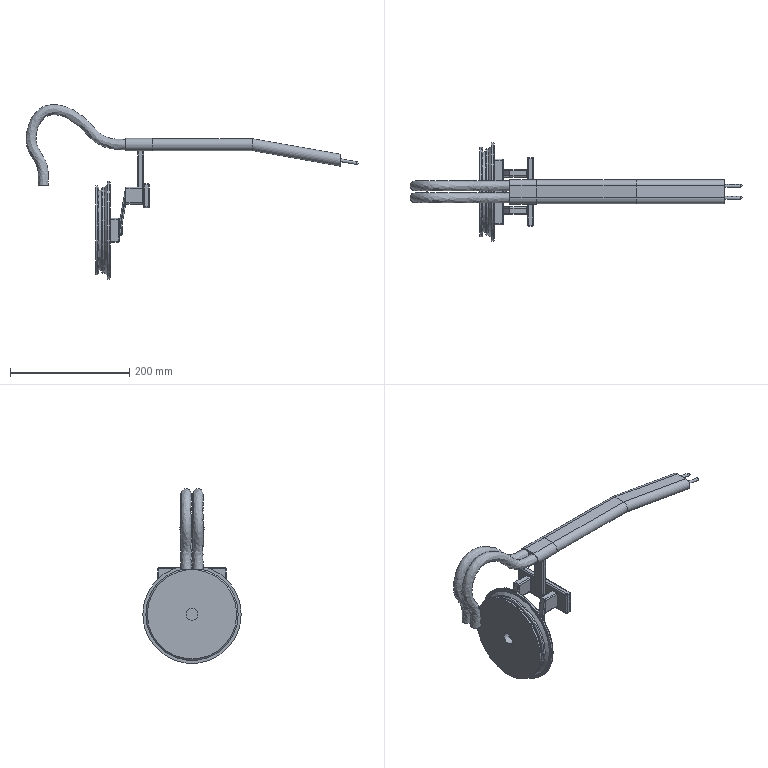Component | NX | 7_NOZZLE | 15 solids | 258 faces | volume 918297 mm3 | plane 138 | cylinder 71 | sphere 20 | torus 11 | spline 10 | other 6 | cone 2 | commonest cylinder face diameters 4 x49 1 x8 20 x3 10 x3 21 x2 5 x2 165 x1 145 x1